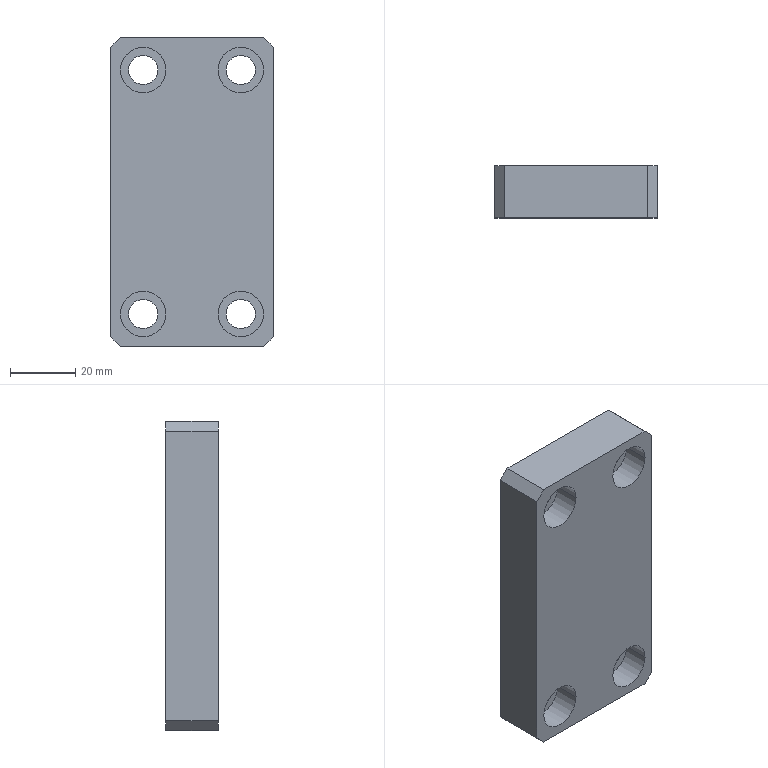Component | SolidWorks | -LowerStopBlock-1 | 1 solid | 30 faces | box 50 x 16 x 95 mm | volume 68750 mm3 | cylinder 16 | plane 14 | commonest cylinder face diameters 14 x8 9 x8
build123d program:
from build123d import *

# Parameters (mm, degrees)
SKETCH1_W                                         = 95
SKETCH1_H                                         = 50
BOSS_EXTRUDE1_DEPTH                               = 8
HOLE_SIZE_ACCORDING_TO_SLOTTED_PAN_HE_D           = 9
HOLE_SIZE_ACCORDING_TO_SLOTTED_PAN_HE_CBORE_D     = 14
HOLE_SIZE_ACCORDING_TO_SLOTTED_PAN_HE_CBORE_DEPTH = 8
CHAMFER1_SIZE                                     = 3


with BuildPart() as part:
    # Sketch1 → Boss-Extrude1 (new, symmetric)
    with BuildSketch(Plane(origin=(0, 0, 0), x_dir=(1, 0, 0), z_dir=(0, 1, 0))):
        Rectangle(SKETCH1_W, SKETCH1_H)
    extrude(amount=BOSS_EXTRUDE1_DEPTH, both=True)

    # Hole Size _ according to_ Slotted Pan He (through all)
    with Locations(Plane(origin=(0, 8, 0), x_dir=(1, 0, 0), z_dir=(0, 1, 0))):
        with Locations((-37.5, 15), (-37.5, -15), (37.5, 15), (37.5, -15)):
            CounterBoreHole(HOLE_SIZE_ACCORDING_TO_SLOTTED_PAN_HE_D / 2, HOLE_SIZE_ACCORDING_TO_SLOTTED_PAN_HE_CBORE_D / 2, HOLE_SIZE_ACCORDING_TO_SLOTTED_PAN_HE_CBORE_DEPTH)

    # Chamfer1
    chamfer1_edges = [part.edges().sort_by_distance(p)[0] for p in [
        (-47.5, 0, -25),
        (47.5, 0, -25),
        (47.5, 0, 25),
        (-47.5, 0, 25),
    ]]
    chamfer(chamfer1_edges, length=CHAMFER1_SIZE)


solid = part.part

# Placed as in the assembly
solid = solid.moved(Location((30, 1036.5, -40), (180, 90, 0)))
STEP:
#1=CARTESIAN_POINT('',(2.047,40.807,-0.09843));
#2=VERTEX_POINT('',#1);
#3=CARTESIAN_POINT('',(1.496,40.807,-0.09843));
#4=VERTEX_POINT('',#3);
#5=CARTESIAN_POINT('',(1.772,40.807,-0.09843));
#6=DIRECTION('',(0.,-1.,0.));
#7=DIRECTION('',(-1.,0.,-0.));
#8=AXIS2_PLACEMENT_3D('',#5,#6,#7);
#9=CIRCLE('',#8,0.2756);
#10=EDGE_CURVE('',#2,#4,#9,.T.);
#11=ORIENTED_EDGE('',*,*,#10,.F.);
#12=CARTESIAN_POINT('',(2.047,40.492,-0.09843));
#13=VERTEX_POINT('',#12);
#14=CARTESIAN_POINT('',(2.047,40.492,-0.09843));
#15=DIRECTION('',(0.,-1.,0.));
#16=VECTOR('',#15,39.37);
#17=LINE('',#14,#16);
#18=EDGE_CURVE('',#2,#13,#17,.T.);
#19=ORIENTED_EDGE('',*,*,#18,.T.);
#20=CARTESIAN_POINT('',(1.496,40.492,-0.09843));
#21=VERTEX_POINT('',#20);
#22=CARTESIAN_POINT('',(1.772,40.492,-0.09843));
#23=DIRECTION('',(0.,-1.,0.));
#24=DIRECTION('',(-1.,0.,-0.));
#25=AXIS2_PLACEMENT_3D('',#22,#23,#24);
#26=CIRCLE('',#25,0.2756);
#27=EDGE_CURVE('',#13,#21,#26,.T.);
#28=ORIENTED_EDGE('',*,*,#27,.T.);
#29=CARTESIAN_POINT('',(1.496,40.492,-0.09843));
#30=DIRECTION('',(0.,-1.,0.));
#31=VECTOR('',#30,39.37);
#32=LINE('',#29,#31);
#33=EDGE_CURVE('',#4,#21,#32,.T.);
#34=ORIENTED_EDGE('',*,*,#33,.F.);
#35=EDGE_LOOP('',(#11,#19,#28,#34));
#36=FACE_OUTER_BOUND('',#35,.T.);
#37=CARTESIAN_POINT('',(1.772,40.492,-0.09843));
#38=DIRECTION('',(0.,-1.,0.));
#39=DIRECTION('',(-1.,0.,-0.));
#40=AXIS2_PLACEMENT_3D('',#37,#38,#39);
#41=CYLINDRICAL_SURFACE('',#40,0.2756);
#42=ADVANCED_FACE('',(#36),#41,.F.);
#43=CARTESIAN_POINT('',(1.949,41.122,-0.09843));
#44=VERTEX_POINT('',#43);
#45=CARTESIAN_POINT('',(1.594,41.122,-0.09843));
#46=VERTEX_POINT('',#45);
#47=CARTESIAN_POINT('',(1.772,41.122,-0.09843));
#48=DIRECTION('',(0.,-1.,0.));
#49=DIRECTION('',(-1.,0.,-0.));
#50=AXIS2_PLACEMENT_3D('',#47,#48,#49);
#51=CIRCLE('',#50,0.1772);
#52=EDGE_CURVE('',#44,#46,#51,.T.);
#53=ORIENTED_EDGE('',*,*,#52,.F.);
#54=CARTESIAN_POINT('',(1.949,40.807,-0.09843));
#55=VERTEX_POINT('',#54);
#56=CARTESIAN_POINT('',(1.949,40.492,-0.09843));
#57=DIRECTION('',(0.,-1.,0.));
#58=VECTOR('',#57,39.37);
#59=LINE('',#56,#58);
#60=EDGE_CURVE('',#44,#55,#59,.T.);
#61=ORIENTED_EDGE('',*,*,#60,.T.);
#62=CARTESIAN_POINT('',(1.594,40.807,-0.09843));
#63=VERTEX_POINT('',#62);
#64=CARTESIAN_POINT('',(1.772,40.807,-0.09843));
#65=DIRECTION('',(0.,-1.,0.));
#66=DIRECTION('',(-1.,0.,-0.));
#67=AXIS2_PLACEMENT_3D('',#64,#65,#66);
#68=CIRCLE('',#67,0.1772);
#69=EDGE_CURVE('',#55,#63,#68,.T.);
#70=ORIENTED_EDGE('',*,*,#69,.T.);
#71=CARTESIAN_POINT('',(1.594,40.492,-0.09843));
#72=DIRECTION('',(0.,-1.,0.));
#73=VECTOR('',#72,39.37);
#74=LINE('',#71,#73);
#75=EDGE_CURVE('',#46,#63,#74,.T.);
#76=ORIENTED_EDGE('',*,*,#75,.F.);
#77=EDGE_LOOP('',(#53,#61,#70,#76));
#78=FACE_OUTER_BOUND('',#77,.T.);
#79=CARTESIAN_POINT('',(1.772,40.492,-0.09843));
#80=DIRECTION('',(0.,-1.,0.));
#81=DIRECTION('',(-1.,0.,-0.));
#82=AXIS2_PLACEMENT_3D('',#79,#80,#81);
#83=CYLINDRICAL_SURFACE('',#82,0.1772);
#84=ADVANCED_FACE('',(#78),#83,.F.);
#85=CARTESIAN_POINT('',(0.8661,40.807,-0.09843));
#86=VERTEX_POINT('',#85);
#87=CARTESIAN_POINT('',(0.315,40.807,-0.09843));
#88=VERTEX_POINT('',#87);
#89=CARTESIAN_POINT('',(0.5906,40.807,-0.09843));
#90=DIRECTION('',(0.,-1.,0.));
#91=DIRECTION('',(-1.,0.,-0.));
#92=AXIS2_PLACEMENT_3D('',#89,#90,#91);
#93=CIRCLE('',#92,0.2756);
#94=EDGE_CURVE('',#86,#88,#93,.T.);
#95=ORIENTED_EDGE('',*,*,#94,.F.);
#96=CARTESIAN_POINT('',(0.8661,40.492,-0.09843));
#97=VERTEX_POINT('',#96);
#98=CARTESIAN_POINT('',(0.8661,40.492,-0.09843));
#99=DIRECTION('',(0.,-1.,0.));
#100=VECTOR('',#99,39.37);
#101=LINE('',#98,#100);
#102=EDGE_CURVE('',#86,#97,#101,.T.);
#103=ORIENTED_EDGE('',*,*,#102,.T.);
#104=CARTESIAN_POINT('',(0.315,40.492,-0.09843));
#105=VERTEX_POINT('',#104);
#106=CARTESIAN_POINT('',(0.5906,40.492,-0.09843));
#107=DIRECTION('',(0.,-1.,0.));
#108=DIRECTION('',(-1.,0.,-0.));
#109=AXIS2_PLACEMENT_3D('',#106,#107,#108);
#110=CIRCLE('',#109,0.2756);
#111=EDGE_CURVE('',#97,#105,#110,.T.);
#112=ORIENTED_EDGE('',*,*,#111,.T.);
#113=CARTESIAN_POINT('',(0.315,40.492,-0.09843));
#114=DIRECTION('',(0.,-1.,0.));
#115=VECTOR('',#114,39.37);
#116=LINE('',#113,#115);
#117=EDGE_CURVE('',#88,#105,#116,.T.);
#118=ORIENTED_EDGE('',*,*,#117,.F.);
#119=EDGE_LOOP('',(#95,#103,#112,#118));
#120=FACE_OUTER_BOUND('',#119,.T.);
#121=CARTESIAN_POINT('',(0.5906,40.492,-0.09843));
#122=DIRECTION('',(0.,-1.,0.));
#123=DIRECTION('',(-1.,0.,-0.));
#124=AXIS2_PLACEMENT_3D('',#121,#122,#123);
#125=CYLINDRICAL_SURFACE('',#124,0.2756);
#126=ADVANCED_FACE('',(#120),#125,.F.);
#127=CARTESIAN_POINT('',(0.7677,41.122,-0.09843));
#128=VERTEX_POINT('',#127);
#129=CARTESIAN_POINT('',(0.4134,41.122,-0.09843));
#130=VERTEX_POINT('',#129);
#131=CARTESIAN_POINT('',(0.5906,41.122,-0.09843));
#132=DIRECTION('',(0.,-1.,0.));
#133=DIRECTION('',(-1.,0.,-0.));
#134=AXIS2_PLACEMENT_3D('',#131,#132,#133);
#135=CIRCLE('',#134,0.1772);
#136=EDGE_CURVE('',#128,#130,#135,.T.);
#137=ORIENTED_EDGE('',*,*,#136,.F.);
#138=CARTESIAN_POINT('',(0.7677,40.807,-0.09843));
#139=VERTEX_POINT('',#138);
#140=CARTESIAN_POINT('',(0.7677,40.492,-0.09843));
#141=DIRECTION('',(0.,-1.,0.));
#142=VECTOR('',#141,39.37);
#143=LINE('',#140,#142);
#144=EDGE_CURVE('',#128,#139,#143,.T.);
#145=ORIENTED_EDGE('',*,*,#144,.T.);
#146=CARTESIAN_POINT('',(0.4134,40.807,-0.09843));
#147=VERTEX_POINT('',#146);
#148=CARTESIAN_POINT('',(0.5906,40.807,-0.09843));
#149=DIRECTION('',(0.,-1.,0.));
#150=DIRECTION('',(-1.,0.,-0.));
#151=AXIS2_PLACEMENT_3D('',#148,#149,#150);
#152=CIRCLE('',#151,0.1772);
#153=EDGE_CURVE('',#139,#147,#152,.T.);
#154=ORIENTED_EDGE('',*,*,#153,.T.);
#155=CARTESIAN_POINT('',(0.4134,40.492,-0.09843));
#156=DIRECTION('',(0.,-1.,0.));
#157=VECTOR('',#156,39.37);
#158=LINE('',#155,#157);
#159=EDGE_CURVE('',#130,#147,#158,.T.);
#160=ORIENTED_EDGE('',*,*,#159,.F.);
#161=EDGE_LOOP('',(#137,#145,#154,#160));
#162=FACE_OUTER_BOUND('',#161,.T.);
#163=CARTESIAN_POINT('',(0.5906,40.492,-0.09843));
#164=DIRECTION('',(0.,-1.,0.));
#165=DIRECTION('',(-1.,0.,-0.));
#166=AXIS2_PLACEMENT_3D('',#163,#164,#165);
#167=CYLINDRICAL_SURFACE('',#166,0.1772);
#168=ADVANCED_FACE('',(#162),#167,.F.);
#169=CARTESIAN_POINT('',(2.047,40.807,-3.051));
#170=VERTEX_POINT('',#169);
#171=CARTESIAN_POINT('',(1.496,40.807,-3.051));
#172=VERTEX_POINT('',#171);
#173=CARTESIAN_POINT('',(1.772,40.807,-3.051));
#174=DIRECTION('',(0.,-1.,0.));
#175=DIRECTION('',(-1.,0.,0.));
#176=AXIS2_PLACEMENT_3D('',#173,#174,#175);
#177=CIRCLE('',#176,0.2756);
#178=EDGE_CURVE('',#170,#172,#177,.T.);
#179=ORIENTED_EDGE('',*,*,#178,.F.);
#180=CARTESIAN_POINT('',(2.047,40.492,-3.051));
#181=VERTEX_POINT('',#180);
#182=CARTESIAN_POINT('',(2.047,40.492,-3.051));
#183=DIRECTION('',(0.,-1.,0.));
#184=VECTOR('',#183,39.37);
#185=LINE('',#182,#184);
#186=EDGE_CURVE('',#170,#181,#185,.T.);
#187=ORIENTED_EDGE('',*,*,#186,.T.);
#188=CARTESIAN_POINT('',(1.496,40.492,-3.051));
#189=VERTEX_POINT('',#188);
#190=CARTESIAN_POINT('',(1.772,40.492,-3.051));
#191=DIRECTION('',(0.,-1.,0.));
#192=DIRECTION('',(-1.,0.,0.));
#193=AXIS2_PLACEMENT_3D('',#190,#191,#192);
#194=CIRCLE('',#193,0.2756);
#195=EDGE_CURVE('',#181,#189,#194,.T.);
#196=ORIENTED_EDGE('',*,*,#195,.T.);
#197=CARTESIAN_POINT('',(1.496,40.492,-3.051));
#198=DIRECTION('',(0.,-1.,0.));
#199=VECTOR('',#198,39.37);
#200=LINE('',#197,#199);
#201=EDGE_CURVE('',#172,#189,#200,.T.);
#202=ORIENTED_EDGE('',*,*,#201,.F.);
#203=EDGE_LOOP('',(#179,#187,#196,#202));
#204=FACE_OUTER_BOUND('',#203,.T.);
#205=CARTESIAN_POINT('',(1.772,40.492,-3.051));
#206=DIRECTION('',(0.,-1.,0.));
#207=DIRECTION('',(-1.,0.,0.));
#208=AXIS2_PLACEMENT_3D('',#205,#206,#207);
#209=CYLINDRICAL_SURFACE('',#208,0.2756);
#210=ADVANCED_FACE('',(#204),#209,.F.);
#211=CARTESIAN_POINT('',(1.949,41.122,-3.051));
#212=VERTEX_POINT('',#211);
#213=CARTESIAN_POINT('',(1.594,41.122,-3.051));
#214=VERTEX_POINT('',#213);
#215=CARTESIAN_POINT('',(1.772,41.122,-3.051));
#216=DIRECTION('',(0.,-1.,0.));
#217=DIRECTION('',(-1.,0.,0.));
#218=AXIS2_PLACEMENT_3D('',#215,#216,#217);
#219=CIRCLE('',#218,0.1772);
#220=EDGE_CURVE('',#212,#214,#219,.T.);
#221=ORIENTED_EDGE('',*,*,#220,.F.);
#222=CARTESIAN_POINT('',(1.949,40.807,-3.051));
#223=VERTEX_POINT('',#222);
#224=CARTESIAN_POINT('',(1.949,40.492,-3.051));
#225=DIRECTION('',(0.,-1.,0.));
#226=VECTOR('',#225,39.37);
#227=LINE('',#224,#226);
#228=EDGE_CURVE('',#212,#223,#227,.T.);
#229=ORIENTED_EDGE('',*,*,#228,.T.);
#230=CARTESIAN_POINT('',(1.594,40.807,-3.051));
#231=VERTEX_POINT('',#230);
#232=CARTESIAN_POINT('',(1.772,40.807,-3.051));
#233=DIRECTION('',(0.,-1.,0.));
#234=DIRECTION('',(-1.,0.,0.));
#235=AXIS2_PLACEMENT_3D('',#232,#233,#234);
#236=CIRCLE('',#235,0.1772);
#237=EDGE_CURVE('',#223,#231,#236,.T.);
#238=ORIENTED_EDGE('',*,*,#237,.T.);
#239=CARTESIAN_POINT('',(1.594,40.492,-3.051));
#240=DIRECTION('',(0.,-1.,0.));
#241=VECTOR('',#240,39.37);
#242=LINE('',#239,#241);
#243=EDGE_CURVE('',#214,#231,#242,.T.);
#244=ORIENTED_EDGE('',*,*,#243,.F.);
#245=EDGE_LOOP('',(#221,#229,#238,#244));
#246=FACE_OUTER_BOUND('',#245,.T.);
#247=CARTESIAN_POINT('',(1.772,40.492,-3.051));
#248=DIRECTION('',(0.,-1.,0.));
#249=DIRECTION('',(-1.,0.,0.));
#250=AXIS2_PLACEMENT_3D('',#247,#248,#249);
#251=CYLINDRICAL_SURFACE('',#250,0.1772);
#252=ADVANCED_FACE('',(#246),#251,.F.);
#253=CARTESIAN_POINT('',(0.8661,40.807,-3.051));
#254=VERTEX_POINT('',#253);
#255=CARTESIAN_POINT('',(0.315,40.807,-3.051));
#256=VERTEX_POINT('',#255);
#257=CARTESIAN_POINT('',(0.5906,40.807,-3.051));
#258=DIRECTION('',(0.,-1.,0.));
#259=DIRECTION('',(-1.,0.,0.));
#260=AXIS2_PLACEMENT_3D('',#257,#258,#259);
#261=CIRCLE('',#260,0.2756);
#262=EDGE_CURVE('',#254,#256,#261,.T.);
#263=ORIENTED_EDGE('',*,*,#262,.F.);
#264=CARTESIAN_POINT('',(0.8661,40.492,-3.051));
#265=VERTEX_POINT('',#264);
#266=CARTESIAN_POINT('',(0.8661,40.492,-3.051));
#267=DIRECTION('',(0.,-1.,0.));
#268=VECTOR('',#267,39.37);
#269=LINE('',#266,#268);
#270=EDGE_CURVE('',#254,#265,#269,.T.);
#271=ORIENTED_EDGE('',*,*,#270,.T.);
#272=CARTESIAN_POINT('',(0.315,40.492,-3.051));
#273=VERTEX_POINT('',#272);
#274=CARTESIAN_POINT('',(0.5906,40.492,-3.051));
#275=DIRECTION('',(0.,-1.,0.));
#276=DIRECTION('',(-1.,0.,0.));
#277=AXIS2_PLACEMENT_3D('',#274,#275,#276);
#278=CIRCLE('',#277,0.2756);
#279=EDGE_CURVE('',#265,#273,#278,.T.);
#280=ORIENTED_EDGE('',*,*,#279,.T.);
#281=CARTESIAN_POINT('',(0.315,40.492,-3.051));
#282=DIRECTION('',(0.,-1.,0.));
#283=VECTOR('',#282,39.37);
#284=LINE('',#281,#283);
#285=EDGE_CURVE('',#256,#273,#284,.T.);
#286=ORIENTED_EDGE('',*,*,#285,.F.);
#287=EDGE_LOOP('',(#263,#271,#280,#286));
#288=FACE_OUTER_BOUND('',#287,.T.);
#289=CARTESIAN_POINT('',(0.5906,40.492,-3.051));
#290=DIRECTION('',(0.,-1.,0.));
#291=DIRECTION('',(-1.,0.,0.));
#292=AXIS2_PLACEMENT_3D('',#289,#290,#291);
#293=CYLINDRICAL_SURFACE('',#292,0.2756);
#294=ADVANCED_FACE('',(#288),#293,.F.);
#295=CARTESIAN_POINT('',(0.7677,41.122,-3.051));
#296=VERTEX_POINT('',#295);
#297=CARTESIAN_POINT('',(0.4134,41.122,-3.051));
#298=VERTEX_POINT('',#297);
#299=CARTESIAN_POINT('',(0.5906,41.122,-3.051));
#300=DIRECTION('',(0.,-1.,0.));
#301=DIRECTION('',(-1.,0.,0.));
#302=AXIS2_PLACEMENT_3D('',#299,#300,#301);
#303=CIRCLE('',#302,0.1772);
#304=EDGE_CURVE('',#296,#298,#303,.T.);
#305=ORIENTED_EDGE('',*,*,#304,.F.);
#306=CARTESIAN_POINT('',(0.7677,40.807,-3.051));
#307=VERTEX_POINT('',#306);
#308=CARTESIAN_POINT('',(0.7677,40.492,-3.051));
#309=DIRECTION('',(0.,-1.,0.));
#310=VECTOR('',#309,39.37);
#311=LINE('',#308,#310);
#312=EDGE_CURVE('',#296,#307,#311,.T.);
#313=ORIENTED_EDGE('',*,*,#312,.T.);
#314=CARTESIAN_POINT('',(0.4134,40.807,-3.051));
#315=VERTEX_POINT('',#314);
#316=CARTESIAN_POINT('',(0.5906,40.807,-3.051));
#317=DIRECTION('',(0.,-1.,0.));
#318=DIRECTION('',(-1.,0.,0.));
#319=AXIS2_PLACEMENT_3D('',#316,#317,#318);
#320=CIRCLE('',#319,0.1772);
#321=EDGE_CURVE('',#307,#315,#320,.T.);
#322=ORIENTED_EDGE('',*,*,#321,.T.);
#323=CARTESIAN_POINT('',(0.4134,40.492,-3.051));
#324=DIRECTION('',(0.,-1.,0.));
#325=VECTOR('',#324,39.37);
#326=LINE('',#323,#325);
#327=EDGE_CURVE('',#298,#315,#326,.T.);
#328=ORIENTED_EDGE('',*,*,#327,.F.);
#329=EDGE_LOOP('',(#305,#313,#322,#328));
#330=FACE_OUTER_BOUND('',#329,.T.);
#331=CARTESIAN_POINT('',(0.5906,40.492,-3.051));
#332=DIRECTION('',(0.,-1.,0.));
#333=DIRECTION('',(-1.,0.,0.));
#334=AXIS2_PLACEMENT_3D('',#331,#332,#333);
#335=CYLINDRICAL_SURFACE('',#334,0.1772);
#336=ADVANCED_FACE('',(#330),#335,.F.);
#337=CARTESIAN_POINT('',(2.047,40.492,0.2953));
#338=VERTEX_POINT('',#337);
#339=CARTESIAN_POINT('',(0.315,40.492,0.2953));
#340=VERTEX_POINT('',#339);
#341=CARTESIAN_POINT('',(0.1969,40.492,0.2953));
#342=DIRECTION('',(-1.,0.,-0.));
#343=VECTOR('',#342,39.37);
#344=LINE('',#341,#343);
#345=EDGE_CURVE('',#338,#340,#344,.T.);
#346=ORIENTED_EDGE('',*,*,#345,.F.);
#347=CARTESIAN_POINT('',(2.047,41.122,0.2953));
#348=VERTEX_POINT('',#347);
#349=CARTESIAN_POINT('',(2.047,40.492,0.2953));
#350=DIRECTION('',(0.,1.,0.));
#351=VECTOR('',#350,39.37);
#352=LINE('',#349,#351);
#353=EDGE_CURVE('',#338,#348,#352,.T.);
#354=ORIENTED_EDGE('',*,*,#353,.T.);
#355=CARTESIAN_POINT('',(0.315,41.122,0.2953));
#356=VERTEX_POINT('',#355);
#357=CARTESIAN_POINT('',(0.1969,41.122,0.2953));
#358=DIRECTION('',(-1.,0.,-0.));
#359=VECTOR('',#358,39.37);
#360=LINE('',#357,#359);
#361=EDGE_CURVE('',#348,#356,#360,.T.);
#362=ORIENTED_EDGE('',*,*,#361,.T.);
#363=CARTESIAN_POINT('',(0.315,40.492,0.2953));
#364=DIRECTION('',(0.,-1.,0.));
#365=VECTOR('',#364,39.37);
#366=LINE('',#363,#365);
#367=EDGE_CURVE('',#356,#340,#366,.T.);
#368=ORIENTED_EDGE('',*,*,#367,.T.);
#369=EDGE_LOOP('',(#346,#354,#362,#368));
#370=FACE_OUTER_BOUND('',#369,.T.);
#371=CARTESIAN_POINT('',(0.1969,40.492,0.2953));
#372=DIRECTION('',(0.,0.,-1.));
#373=DIRECTION('',(1.,0.,0.));
#374=AXIS2_PLACEMENT_3D('',#371,#372,#373);
#375=PLANE('',#374);
#376=ADVANCED_FACE('',(#370),#375,.F.);
#377=CARTESIAN_POINT('',(0.1969,41.122,0.1772));
#378=VERTEX_POINT('',#377);
#379=CARTESIAN_POINT('',(0.1969,41.122,-3.327));
#380=VERTEX_POINT('',#379);
#381=CARTESIAN_POINT('',(0.1969,41.122,-3.445));
#382=DIRECTION('',(0.,0.,-1.));
#383=VECTOR('',#382,39.37);
#384=LINE('',#381,#383);
#385=EDGE_CURVE('',#378,#380,#384,.T.);
#386=ORIENTED_EDGE('',*,*,#385,.T.);
#387=CARTESIAN_POINT('',(0.1969,40.492,-3.327));
#388=VERTEX_POINT('',#387);
#389=CARTESIAN_POINT('',(0.1969,40.492,-3.327));
#390=DIRECTION('',(0.,-1.,0.));
#391=VECTOR('',#390,39.37);
#392=LINE('',#389,#391);
#393=EDGE_CURVE('',#380,#388,#392,.T.);
#394=ORIENTED_EDGE('',*,*,#393,.T.);
#395=CARTESIAN_POINT('',(0.1969,40.492,0.1772));
#396=VERTEX_POINT('',#395);
#397=CARTESIAN_POINT('',(0.1969,40.492,-3.445));
#398=DIRECTION('',(0.,0.,-1.));
#399=VECTOR('',#398,39.37);
#400=LINE('',#397,#399);
#401=EDGE_CURVE('',#396,#388,#400,.T.);
#402=ORIENTED_EDGE('',*,*,#401,.F.);
#403=CARTESIAN_POINT('',(0.1969,40.492,0.1772));
#404=DIRECTION('',(0.,1.,0.));
#405=VECTOR('',#404,39.37);
#406=LINE('',#403,#405);
#407=EDGE_CURVE('',#396,#378,#406,.T.);
#408=ORIENTED_EDGE('',*,*,#407,.T.);
#409=EDGE_LOOP('',(#386,#394,#402,#408));
#410=FACE_OUTER_BOUND('',#409,.T.);
#411=CARTESIAN_POINT('',(0.1969,40.492,-3.445));
#412=DIRECTION('',(1.,0.,0.));
#413=DIRECTION('',(-0.,0.,1.));
#414=AXIS2_PLACEMENT_3D('',#411,#412,#413);
#415=PLANE('',#414);
#416=ADVANCED_FACE('',(#410),#415,.F.);
#417=CARTESIAN_POINT('',(0.315,40.492,-3.445));
#418=VERTEX_POINT('',#417);
#419=CARTESIAN_POINT('',(2.047,40.492,-3.445));
#420=VERTEX_POINT('',#419);
#421=CARTESIAN_POINT('',(0.1969,40.492,-3.445));
#422=DIRECTION('',(1.,0.,0.));
#423=VECTOR('',#422,39.37);
#424=LINE('',#421,#423);
#425=EDGE_CURVE('',#418,#420,#424,.T.);
#426=ORIENTED_EDGE('',*,*,#425,.F.);
#427=CARTESIAN_POINT('',(0.315,41.122,-3.445));
#428=VERTEX_POINT('',#427);
#429=CARTESIAN_POINT('',(0.315,40.492,-3.445));
#430=DIRECTION('',(0.,1.,0.));
#431=VECTOR('',#430,39.37);
#432=LINE('',#429,#431);
#433=EDGE_CURVE('',#418,#428,#432,.T.);
#434=ORIENTED_EDGE('',*,*,#433,.T.);
#435=CARTESIAN_POINT('',(2.047,41.122,-3.445));
#436=VERTEX_POINT('',#435);
#437=CARTESIAN_POINT('',(0.1969,41.122,-3.445));
#438=DIRECTION('',(1.,0.,0.));
#439=VECTOR('',#438,39.37);
#440=LINE('',#437,#439);
#441=EDGE_CURVE('',#428,#436,#440,.T.);
#442=ORIENTED_EDGE('',*,*,#441,.T.);
#443=CARTESIAN_POINT('',(2.047,40.492,-3.445));
#444=DIRECTION('',(0.,-1.,0.));
#445=VECTOR('',#444,39.37);
#446=LINE('',#443,#445);
#447=EDGE_CURVE('',#436,#420,#446,.T.);
#448=ORIENTED_EDGE('',*,*,#447,.T.);
#449=EDGE_LOOP('',(#426,#434,#442,#448));
#450=FACE_OUTER_BOUND('',#449,.T.);
#451=CARTESIAN_POINT('',(0.1969,40.492,-3.445));
#452=DIRECTION('',(-0.,0.,1.));
#453=DIRECTION('',(-1.,0.,-0.));
#454=AXIS2_PLACEMENT_3D('',#451,#452,#453);
#455=PLANE('',#454);
#456=ADVANCED_FACE('',(#450),#455,.F.);
#457=CARTESIAN_POINT('',(2.165,40.492,-3.327));
#458=VERTEX_POINT('',#457);
#459=CARTESIAN_POINT('',(2.165,40.492,0.1772));
#460=VERTEX_POINT('',#459);
#461=CARTESIAN_POINT('',(2.165,40.492,-3.445));
#462=DIRECTION('',(-0.,0.,1.));
#463=VECTOR('',#462,39.37);
#464=LINE('',#461,#463);
#465=EDGE_CURVE('',#458,#460,#464,.T.);
#466=ORIENTED_EDGE('',*,*,#465,.F.);
#467=CARTESIAN_POINT('',(2.165,41.122,-3.327));
#468=VERTEX_POINT('',#467);
#469=CARTESIAN_POINT('',(2.165,40.492,-3.327));
#470=DIRECTION('',(0.,1.,0.));
#471=VECTOR('',#470,39.37);
#472=LINE('',#469,#471);
#473=EDGE_CURVE('',#458,#468,#472,.T.);
#474=ORIENTED_EDGE('',*,*,#473,.T.);
#475=CARTESIAN_POINT('',(2.165,41.122,0.1772));
#476=VERTEX_POINT('',#475);
#477=CARTESIAN_POINT('',(2.165,41.122,-3.445));
#478=DIRECTION('',(-0.,0.,1.));
#479=VECTOR('',#478,39.37);
#480=LINE('',#477,#479);
#481=EDGE_CURVE('',#468,#476,#480,.T.);
#482=ORIENTED_EDGE('',*,*,#481,.T.);
#483=CARTESIAN_POINT('',(2.165,40.492,0.1772));
#484=DIRECTION('',(0.,-1.,0.));
#485=VECTOR('',#484,39.37);
#486=LINE('',#483,#485);
#487=EDGE_CURVE('',#476,#460,#486,.T.);
#488=ORIENTED_EDGE('',*,*,#487,.T.);
#489=EDGE_LOOP('',(#466,#474,#482,#488));
#490=FACE_OUTER_BOUND('',#489,.T.);
#491=CARTESIAN_POINT('',(2.165,40.492,-3.445));
#492=DIRECTION('',(-1.,0.,-0.));
#493=DIRECTION('',(0.,0.,-1.));
#494=AXIS2_PLACEMENT_3D('',#491,#492,#493);
#495=PLANE('',#494);
#496=ADVANCED_FACE('',(#490),#495,.F.);
#497=CARTESIAN_POINT('',(1.772,40.492,-0.09843));
#498=DIRECTION('',(0.,-1.,0.));
#499=DIRECTION('',(-1.,0.,-0.));
#500=AXIS2_PLACEMENT_3D('',#497,#498,#499);
#501=CIRCLE('',#500,0.2756);
#502=EDGE_CURVE('',#21,#13,#501,.T.);
#503=ORIENTED_EDGE('',*,*,#502,.F.);
#504=ORIENTED_EDGE('',*,*,#27,.F.);
#505=EDGE_LOOP('',(#503,#504));
#506=FACE_BOUND('',#505,.T.);
#507=CARTESIAN_POINT('',(0.5906,40.492,-0.09843));
#508=DIRECTION('',(0.,-1.,0.));
#509=DIRECTION('',(-1.,0.,-0.));
#510=AXIS2_PLACEMENT_3D('',#507,#508,#509);
#511=CIRCLE('',#510,0.2756);
#512=EDGE_CURVE('',#105,#97,#511,.T.);
#513=ORIENTED_EDGE('',*,*,#512,.F.);
#514=ORIENTED_EDGE('',*,*,#111,.F.);
#515=EDGE_LOOP('',(#513,#514));
#516=FACE_BOUND('',#515,.T.);
#517=CARTESIAN_POINT('',(1.772,40.492,-3.051));
#518=DIRECTION('',(0.,-1.,0.));
#519=DIRECTION('',(-1.,0.,0.));
#520=AXIS2_PLACEMENT_3D('',#517,#518,#519);
#521=CIRCLE('',#520,0.2756);
#522=EDGE_CURVE('',#189,#181,#521,.T.);
#523=ORIENTED_EDGE('',*,*,#522,.F.);
#524=ORIENTED_EDGE('',*,*,#195,.F.);
#525=EDGE_LOOP('',(#523,#524));
#526=FACE_BOUND('',#525,.T.);
#527=CARTESIAN_POINT('',(0.5906,40.492,-3.051));
#528=DIRECTION('',(0.,-1.,0.));
#529=DIRECTION('',(-1.,0.,0.));
#530=AXIS2_PLACEMENT_3D('',#527,#528,#529);
#531=CIRCLE('',#530,0.2756);
#532=EDGE_CURVE('',#273,#265,#531,.T.);
#533=ORIENTED_EDGE('',*,*,#532,.F.);
#534=ORIENTED_EDGE('',*,*,#279,.F.);
#535=EDGE_LOOP('',(#533,#534));
#536=FACE_BOUND('',#535,.T.);
#537=ORIENTED_EDGE('',*,*,#401,.T.);
#538=CARTESIAN_POINT('',(-0.187,40.492,-2.943));
#539=DIRECTION('',(0.7071,0.,-0.7071));
#540=VECTOR('',#539,39.37);
#541=LINE('',#538,#540);
#542=EDGE_CURVE('',#388,#418,#541,.T.);
#543=ORIENTED_EDGE('',*,*,#542,.T.);
#544=ORIENTED_EDGE('',*,*,#425,.T.);
#545=CARTESIAN_POINT('',(2.549,40.492,-2.943));
#546=DIRECTION('',(0.7071,0.,0.7071));
#547=VECTOR('',#546,39.37);
#548=LINE('',#545,#547);
#549=EDGE_CURVE('',#420,#458,#548,.T.);
#550=ORIENTED_EDGE('',*,*,#549,.T.);
#551=ORIENTED_EDGE('',*,*,#465,.T.);
#552=CARTESIAN_POINT('',(2.549,40.492,-0.2067));
#553=DIRECTION('',(-0.7071,0.,0.7071));
#554=VECTOR('',#553,39.37);
#555=LINE('',#552,#554);
#556=EDGE_CURVE('',#460,#338,#555,.T.);
#557=ORIENTED_EDGE('',*,*,#556,.T.);
#558=ORIENTED_EDGE('',*,*,#345,.T.);
#559=CARTESIAN_POINT('',(-0.187,40.492,-0.2067));
#560=DIRECTION('',(-0.7071,0.,-0.7071));
#561=VECTOR('',#560,39.37);
#562=LINE('',#559,#561);
#563=EDGE_CURVE('',#340,#396,#562,.T.);
#564=ORIENTED_EDGE('',*,*,#563,.T.);
#565=EDGE_LOOP('',(#537,#543,#544,#550,#551,#557,#558,#564));
#566=FACE_OUTER_BOUND('',#565,.T.);
#567=CARTESIAN_POINT('',(1.181,40.492,-1.575));
#568=DIRECTION('',(0.,-1.,0.));
#569=DIRECTION('',(-1.,0.,-0.));
#570=AXIS2_PLACEMENT_3D('',#567,#568,#569);
#571=PLANE('',#570);
#572=ADVANCED_FACE('',(#506,#516,#526,#536,#566),#571,.T.);
#573=CARTESIAN_POINT('',(1.772,41.122,-0.09843));
#574=DIRECTION('',(0.,-1.,0.));
#575=DIRECTION('',(-1.,0.,-0.));
#576=AXIS2_PLACEMENT_3D('',#573,#574,#575);
#577=CIRCLE('',#576,0.1772);
#578=EDGE_CURVE('',#46,#44,#577,.T.);
#579=ORIENTED_EDGE('',*,*,#578,.T.);
#580=ORIENTED_EDGE('',*,*,#52,.T.);
#581=EDGE_LOOP('',(#579,#580));
#582=FACE_BOUND('',#581,.T.);
#583=CARTESIAN_POINT('',(0.5906,41.122,-0.09843));
#584=DIRECTION('',(0.,-1.,0.));
#585=DIRECTION('',(-1.,0.,-0.));
#586=AXIS2_PLACEMENT_3D('',#583,#584,#585);
#587=CIRCLE('',#586,0.1772);
#588=EDGE_CURVE('',#130,#128,#587,.T.);
#589=ORIENTED_EDGE('',*,*,#588,.T.);
#590=ORIENTED_EDGE('',*,*,#136,.T.);
#591=EDGE_LOOP('',(#589,#590));
#592=FACE_BOUND('',#591,.T.);
#593=CARTESIAN_POINT('',(1.772,41.122,-3.051));
#594=DIRECTION('',(0.,-1.,0.));
#595=DIRECTION('',(-1.,0.,0.));
#596=AXIS2_PLACEMENT_3D('',#593,#594,#595);
#597=CIRCLE('',#596,0.1772);
#598=EDGE_CURVE('',#214,#212,#597,.T.);
#599=ORIENTED_EDGE('',*,*,#598,.T.);
#600=ORIENTED_EDGE('',*,*,#220,.T.);
#601=EDGE_LOOP('',(#599,#600));
#602=FACE_BOUND('',#601,.T.);
#603=CARTESIAN_POINT('',(0.5906,41.122,-3.051));
#604=DIRECTION('',(0.,-1.,0.));
#605=DIRECTION('',(-1.,0.,0.));
#606=AXIS2_PLACEMENT_3D('',#603,#604,#605);
#607=CIRCLE('',#606,0.1772);
#608=EDGE_CURVE('',#298,#296,#607,.T.);
#609=ORIENTED_EDGE('',*,*,#608,.T.);
#610=ORIENTED_EDGE('',*,*,#304,.T.);
#611=EDGE_LOOP('',(#609,#610));
#612=FACE_BOUND('',#611,.T.);
#613=ORIENTED_EDGE('',*,*,#441,.F.);
#614=CARTESIAN_POINT('',(0.315,41.122,-3.445));
#615=DIRECTION('',(-0.7071,0.,0.7071));
#616=VECTOR('',#615,39.37);
#617=LINE('',#614,#616);
#618=EDGE_CURVE('',#428,#380,#617,.T.);
#619=ORIENTED_EDGE('',*,*,#618,.T.);
#620=ORIENTED_EDGE('',*,*,#385,.F.);
#621=CARTESIAN_POINT('',(0.1969,41.122,0.1772));
#622=DIRECTION('',(0.7071,0.,0.7071));
#623=VECTOR('',#622,39.37);
#624=LINE('',#621,#623);
#625=EDGE_CURVE('',#378,#356,#624,.T.);
#626=ORIENTED_EDGE('',*,*,#625,.T.);
#627=ORIENTED_EDGE('',*,*,#361,.F.);
#628=CARTESIAN_POINT('',(2.047,41.122,0.2953));
#629=DIRECTION('',(0.7071,0.,-0.7071));
#630=VECTOR('',#629,39.37);
#631=LINE('',#628,#630);
#632=EDGE_CURVE('',#348,#476,#631,.T.);
#633=ORIENTED_EDGE('',*,*,#632,.T.);
#634=ORIENTED_EDGE('',*,*,#481,.F.);
#635=CARTESIAN_POINT('',(2.165,41.122,-3.327));
#636=DIRECTION('',(-0.7071,0.,-0.7071));
#637=VECTOR('',#636,39.37);
#638=LINE('',#635,#637);
#639=EDGE_CURVE('',#468,#436,#638,.T.);
#640=ORIENTED_EDGE('',*,*,#639,.T.);
#641=EDGE_LOOP('',(#613,#619,#620,#626,#627,#633,#634,#640));
#642=FACE_OUTER_BOUND('',#641,.T.);
#643=CARTESIAN_POINT('',(1.181,41.122,-1.575));
#644=DIRECTION('',(0.,-1.,0.));
#645=DIRECTION('',(-1.,0.,-0.));
#646=AXIS2_PLACEMENT_3D('',#643,#644,#645);
#647=PLANE('',#646);
#648=ADVANCED_FACE('',(#582,#592,#602,#612,#642),#647,.F.);
#649=ORIENTED_EDGE('',*,*,#312,.F.);
#650=ORIENTED_EDGE('',*,*,#608,.F.);
#651=ORIENTED_EDGE('',*,*,#327,.T.);
#652=CARTESIAN_POINT('',(0.5906,40.807,-3.051));
#653=DIRECTION('',(0.,-1.,0.));
#654=DIRECTION('',(-1.,0.,0.));
#655=AXIS2_PLACEMENT_3D('',#652,#653,#654);
#656=CIRCLE('',#655,0.1772);
#657=EDGE_CURVE('',#315,#307,#656,.T.);
#658=ORIENTED_EDGE('',*,*,#657,.T.);
#659=EDGE_LOOP('',(#649,#650,#651,#658));
#660=FACE_OUTER_BOUND('',#659,.T.);
#661=CARTESIAN_POINT('',(0.5906,40.492,-3.051));
#662=DIRECTION('',(0.,-1.,0.));
#663=DIRECTION('',(-1.,0.,0.));
#664=AXIS2_PLACEMENT_3D('',#661,#662,#663);
#665=CYLINDRICAL_SURFACE('',#664,0.1772);
#666=ADVANCED_FACE('',(#660),#665,.F.);
#667=ORIENTED_EDGE('',*,*,#657,.F.);
#668=ORIENTED_EDGE('',*,*,#321,.F.);
#669=EDGE_LOOP('',(#667,#668));
#670=FACE_BOUND('',#669,.T.);
#671=CARTESIAN_POINT('',(0.5906,40.807,-3.051));
#672=DIRECTION('',(0.,-1.,0.));
#673=DIRECTION('',(-1.,0.,0.));
#674=AXIS2_PLACEMENT_3D('',#671,#672,#673);
#675=CIRCLE('',#674,0.2756);
#676=EDGE_CURVE('',#256,#254,#675,.T.);
#677=ORIENTED_EDGE('',*,*,#676,.T.);
#678=ORIENTED_EDGE('',*,*,#262,.T.);
#679=EDGE_LOOP('',(#677,#678));
#680=FACE_OUTER_BOUND('',#679,.T.);
#681=CARTESIAN_POINT('',(0.5906,40.807,-3.228));
#682=DIRECTION('',(0.,1.,0.));
#683=DIRECTION('',(1.,0.,0.));
#684=AXIS2_PLACEMENT_3D('',#681,#682,#683);
#685=PLANE('',#684);
#686=ADVANCED_FACE('',(#670,#680),#685,.F.);
#687=ORIENTED_EDGE('',*,*,#270,.F.);
#688=ORIENTED_EDGE('',*,*,#676,.F.);
#689=ORIENTED_EDGE('',*,*,#285,.T.);
#690=ORIENTED_EDGE('',*,*,#532,.T.);
#691=EDGE_LOOP('',(#687,#688,#689,#690));
#692=FACE_OUTER_BOUND('',#691,.T.);
#693=CARTESIAN_POINT('',(0.5906,40.492,-3.051));
#694=DIRECTION('',(0.,-1.,0.));
#695=DIRECTION('',(-1.,0.,0.));
#696=AXIS2_PLACEMENT_3D('',#693,#694,#695);
#697=CYLINDRICAL_SURFACE('',#696,0.2756);
#698=ADVANCED_FACE('',(#692),#697,.F.);
#699=ORIENTED_EDGE('',*,*,#228,.F.);
#700=ORIENTED_EDGE('',*,*,#598,.F.);
#701=ORIENTED_EDGE('',*,*,#243,.T.);
#702=CARTESIAN_POINT('',(1.772,40.807,-3.051));
#703=DIRECTION('',(0.,-1.,0.));
#704=DIRECTION('',(-1.,0.,0.));
#705=AXIS2_PLACEMENT_3D('',#702,#703,#704);
#706=CIRCLE('',#705,0.1772);
#707=EDGE_CURVE('',#231,#223,#706,.T.);
#708=ORIENTED_EDGE('',*,*,#707,.T.);
#709=EDGE_LOOP('',(#699,#700,#701,#708));
#710=FACE_OUTER_BOUND('',#709,.T.);
#711=CARTESIAN_POINT('',(1.772,40.492,-3.051));
#712=DIRECTION('',(0.,-1.,0.));
#713=DIRECTION('',(-1.,0.,0.));
#714=AXIS2_PLACEMENT_3D('',#711,#712,#713);
#715=CYLINDRICAL_SURFACE('',#714,0.1772);
#716=ADVANCED_FACE('',(#710),#715,.F.);
#717=ORIENTED_EDGE('',*,*,#707,.F.);
#718=ORIENTED_EDGE('',*,*,#237,.F.);
#719=EDGE_LOOP('',(#717,#718));
#720=FACE_BOUND('',#719,.T.);
#721=CARTESIAN_POINT('',(1.772,40.807,-3.051));
#722=DIRECTION('',(0.,-1.,0.));
#723=DIRECTION('',(-1.,0.,0.));
#724=AXIS2_PLACEMENT_3D('',#721,#722,#723);
#725=CIRCLE('',#724,0.2756);
#726=EDGE_CURVE('',#172,#170,#725,.T.);
#727=ORIENTED_EDGE('',*,*,#726,.T.);
#728=ORIENTED_EDGE('',*,*,#178,.T.);
#729=EDGE_LOOP('',(#727,#728));
#730=FACE_OUTER_BOUND('',#729,.T.);
#731=CARTESIAN_POINT('',(1.772,40.807,-3.228));
#732=DIRECTION('',(0.,1.,0.));
#733=DIRECTION('',(1.,0.,0.));
#734=AXIS2_PLACEMENT_3D('',#731,#732,#733);
#735=PLANE('',#734);
#736=ADVANCED_FACE('',(#720,#730),#735,.F.);
#737=ORIENTED_EDGE('',*,*,#186,.F.);
#738=ORIENTED_EDGE('',*,*,#726,.F.);
#739=ORIENTED_EDGE('',*,*,#201,.T.);
#740=ORIENTED_EDGE('',*,*,#522,.T.);
#741=EDGE_LOOP('',(#737,#738,#739,#740));
#742=FACE_OUTER_BOUND('',#741,.T.);
#743=CARTESIAN_POINT('',(1.772,40.492,-3.051));
#744=DIRECTION('',(0.,-1.,0.));
#745=DIRECTION('',(-1.,0.,0.));
#746=AXIS2_PLACEMENT_3D('',#743,#744,#745);
#747=CYLINDRICAL_SURFACE('',#746,0.2756);
#748=ADVANCED_FACE('',(#742),#747,.F.);
#749=ORIENTED_EDGE('',*,*,#144,.F.);
#750=ORIENTED_EDGE('',*,*,#588,.F.);
#751=ORIENTED_EDGE('',*,*,#159,.T.);
#752=CARTESIAN_POINT('',(0.5906,40.807,-0.09843));
#753=DIRECTION('',(0.,-1.,0.));
#754=DIRECTION('',(-1.,0.,-0.));
#755=AXIS2_PLACEMENT_3D('',#752,#753,#754);
#756=CIRCLE('',#755,0.1772);
#757=EDGE_CURVE('',#147,#139,#756,.T.);
#758=ORIENTED_EDGE('',*,*,#757,.T.);
#759=EDGE_LOOP('',(#749,#750,#751,#758));
#760=FACE_OUTER_BOUND('',#759,.T.);
#761=CARTESIAN_POINT('',(0.5906,40.492,-0.09843));
#762=DIRECTION('',(0.,-1.,0.));
#763=DIRECTION('',(-1.,0.,-0.));
#764=AXIS2_PLACEMENT_3D('',#761,#762,#763);
#765=CYLINDRICAL_SURFACE('',#764,0.1772);
#766=ADVANCED_FACE('',(#760),#765,.F.);
#767=ORIENTED_EDGE('',*,*,#757,.F.);
#768=ORIENTED_EDGE('',*,*,#153,.F.);
#769=EDGE_LOOP('',(#767,#768));
#770=FACE_BOUND('',#769,.T.);
#771=CARTESIAN_POINT('',(0.5906,40.807,-0.09843));
#772=DIRECTION('',(0.,-1.,0.));
#773=DIRECTION('',(-1.,0.,-0.));
#774=AXIS2_PLACEMENT_3D('',#771,#772,#773);
#775=CIRCLE('',#774,0.2756);
#776=EDGE_CURVE('',#88,#86,#775,.T.);
#777=ORIENTED_EDGE('',*,*,#776,.T.);
#778=ORIENTED_EDGE('',*,*,#94,.T.);
#779=EDGE_LOOP('',(#777,#778));
#780=FACE_OUTER_BOUND('',#779,.T.);
#781=CARTESIAN_POINT('',(0.5906,40.807,-0.2756));
#782=DIRECTION('',(0.,1.,0.));
#783=DIRECTION('',(1.,0.,0.));
#784=AXIS2_PLACEMENT_3D('',#781,#782,#783);
#785=PLANE('',#784);
#786=ADVANCED_FACE('',(#770,#780),#785,.F.);
#787=ORIENTED_EDGE('',*,*,#102,.F.);
#788=ORIENTED_EDGE('',*,*,#776,.F.);
#789=ORIENTED_EDGE('',*,*,#117,.T.);
#790=ORIENTED_EDGE('',*,*,#512,.T.);
#791=EDGE_LOOP('',(#787,#788,#789,#790));
#792=FACE_OUTER_BOUND('',#791,.T.);
#793=CARTESIAN_POINT('',(0.5906,40.492,-0.09843));
#794=DIRECTION('',(0.,-1.,0.));
#795=DIRECTION('',(-1.,0.,-0.));
#796=AXIS2_PLACEMENT_3D('',#793,#794,#795);
#797=CYLINDRICAL_SURFACE('',#796,0.2756);
#798=ADVANCED_FACE('',(#792),#797,.F.);
#799=ORIENTED_EDGE('',*,*,#60,.F.);
#800=ORIENTED_EDGE('',*,*,#578,.F.);
#801=ORIENTED_EDGE('',*,*,#75,.T.);
#802=CARTESIAN_POINT('',(1.772,40.807,-0.09843));
#803=DIRECTION('',(0.,-1.,0.));
#804=DIRECTION('',(-1.,0.,-0.));
#805=AXIS2_PLACEMENT_3D('',#802,#803,#804);
#806=CIRCLE('',#805,0.1772);
#807=EDGE_CURVE('',#63,#55,#806,.T.);
#808=ORIENTED_EDGE('',*,*,#807,.T.);
#809=EDGE_LOOP('',(#799,#800,#801,#808));
#810=FACE_OUTER_BOUND('',#809,.T.);
#811=CARTESIAN_POINT('',(1.772,40.492,-0.09843));
#812=DIRECTION('',(0.,-1.,0.));
#813=DIRECTION('',(-1.,0.,-0.));
#814=AXIS2_PLACEMENT_3D('',#811,#812,#813);
#815=CYLINDRICAL_SURFACE('',#814,0.1772);
#816=ADVANCED_FACE('',(#810),#815,.F.);
#817=ORIENTED_EDGE('',*,*,#807,.F.);
#818=ORIENTED_EDGE('',*,*,#69,.F.);
#819=EDGE_LOOP('',(#817,#818));
#820=FACE_BOUND('',#819,.T.);
#821=CARTESIAN_POINT('',(1.772,40.807,-0.09843));
#822=DIRECTION('',(0.,-1.,0.));
#823=DIRECTION('',(-1.,0.,-0.));
#824=AXIS2_PLACEMENT_3D('',#821,#822,#823);
#825=CIRCLE('',#824,0.2756);
#826=EDGE_CURVE('',#4,#2,#825,.T.);
#827=ORIENTED_EDGE('',*,*,#826,.T.);
#828=ORIENTED_EDGE('',*,*,#10,.T.);
#829=EDGE_LOOP('',(#827,#828));
#830=FACE_OUTER_BOUND('',#829,.T.);
#831=CARTESIAN_POINT('',(1.772,40.807,-0.2756));
#832=DIRECTION('',(0.,1.,0.));
#833=DIRECTION('',(1.,0.,0.));
#834=AXIS2_PLACEMENT_3D('',#831,#832,#833);
#835=PLANE('',#834);
#836=ADVANCED_FACE('',(#820,#830),#835,.F.);
#837=ORIENTED_EDGE('',*,*,#18,.F.);
#838=ORIENTED_EDGE('',*,*,#826,.F.);
#839=ORIENTED_EDGE('',*,*,#33,.T.);
#840=ORIENTED_EDGE('',*,*,#502,.T.);
#841=EDGE_LOOP('',(#837,#838,#839,#840));
#842=FACE_OUTER_BOUND('',#841,.T.);
#843=CARTESIAN_POINT('',(1.772,40.492,-0.09843));
#844=DIRECTION('',(0.,-1.,0.));
#845=DIRECTION('',(-1.,0.,-0.));
#846=AXIS2_PLACEMENT_3D('',#843,#844,#845);
#847=CYLINDRICAL_SURFACE('',#846,0.2756);
#848=ADVANCED_FACE('',(#842),#847,.F.);
#849=ORIENTED_EDGE('',*,*,#542,.F.);
#850=ORIENTED_EDGE('',*,*,#393,.F.);
#851=ORIENTED_EDGE('',*,*,#618,.F.);
#852=ORIENTED_EDGE('',*,*,#433,.F.);
#853=EDGE_LOOP('',(#849,#850,#851,#852));
#854=FACE_OUTER_BOUND('',#853,.T.);
#855=CARTESIAN_POINT('',(0.315,40.492,-3.445));
#856=DIRECTION('',(0.7071,0.,0.7071));
#857=DIRECTION('',(0.,1.,0.));
#858=AXIS2_PLACEMENT_3D('',#855,#856,#857);
#859=PLANE('',#858);
#860=ADVANCED_FACE('',(#854),#859,.F.);
#861=ORIENTED_EDGE('',*,*,#549,.F.);
#862=ORIENTED_EDGE('',*,*,#447,.F.);
#863=ORIENTED_EDGE('',*,*,#639,.F.);
#864=ORIENTED_EDGE('',*,*,#473,.F.);
#865=EDGE_LOOP('',(#861,#862,#863,#864));
#866=FACE_OUTER_BOUND('',#865,.T.);
#867=CARTESIAN_POINT('',(2.165,40.492,-3.327));
#868=DIRECTION('',(-0.7071,0.,0.7071));
#869=DIRECTION('',(0.,1.,0.));
#870=AXIS2_PLACEMENT_3D('',#867,#868,#869);
#871=PLANE('',#870);
#872=ADVANCED_FACE('',(#866),#871,.F.);
#873=ORIENTED_EDGE('',*,*,#556,.F.);
#874=ORIENTED_EDGE('',*,*,#487,.F.);
#875=ORIENTED_EDGE('',*,*,#632,.F.);
#876=ORIENTED_EDGE('',*,*,#353,.F.);
#877=EDGE_LOOP('',(#873,#874,#875,#876));
#878=FACE_OUTER_BOUND('',#877,.T.);
#879=CARTESIAN_POINT('',(2.047,40.492,0.2953));
#880=DIRECTION('',(-0.7071,0.,-0.7071));
#881=DIRECTION('',(0.,1.,0.));
#882=AXIS2_PLACEMENT_3D('',#879,#880,#881);
#883=PLANE('',#882);
#884=ADVANCED_FACE('',(#878),#883,.F.);
#885=ORIENTED_EDGE('',*,*,#563,.F.);
#886=ORIENTED_EDGE('',*,*,#367,.F.);
#887=ORIENTED_EDGE('',*,*,#625,.F.);
#888=ORIENTED_EDGE('',*,*,#407,.F.);
#889=EDGE_LOOP('',(#885,#886,#887,#888));
#890=FACE_OUTER_BOUND('',#889,.T.);
#891=CARTESIAN_POINT('',(0.1969,40.492,0.1772));
#892=DIRECTION('',(0.7071,0.,-0.7071));
#893=DIRECTION('',(0.,1.,0.));
#894=AXIS2_PLACEMENT_3D('',#891,#892,#893);
#895=PLANE('',#894);
#896=ADVANCED_FACE('',(#890),#895,.F.);
#897=CLOSED_SHELL('',(#42,#84,#126,#168,#210,#252,#294,#336,#376,#416,#456,#496,#572,#648,#666,#686,#698,#716,#736,#748,#766,#786,#798,#816,#836,#848,#860,#872,#884,#896));
#898=MANIFOLD_SOLID_BREP('',#897);
#899=CARTESIAN_POINT('',(0.,0.,0.));
#900=DIRECTION('',(0.,0.,1.));
#901=DIRECTION('',(1.,0.,0.));
#902=AXIS2_PLACEMENT_3D('',#899,#900,#901);
#903=(LENGTH_UNIT()NAMED_UNIT(*)SI_UNIT($,.METRE.));
#904=LENGTH_MEASURE_WITH_UNIT(LENGTH_MEASURE(0.0254),#903);
#905=DIMENSIONAL_EXPONENTS(1.,0.,0.,0.,0.,0.,0.);
#906=(CONVERSION_BASED_UNIT('',#904)LENGTH_UNIT()NAMED_UNIT(#905));
#907=UNCERTAINTY_MEASURE_WITH_UNIT(LENGTH_MEASURE(0.00001),#906,'','');
#908=(NAMED_UNIT(*)PLANE_ANGLE_UNIT()SI_UNIT($,.RADIAN.));
#909=(NAMED_UNIT(*)SI_UNIT($,.STERADIAN.)SOLID_ANGLE_UNIT());
#910=(GEOMETRIC_REPRESENTATION_CONTEXT(3)GLOBAL_UNCERTAINTY_ASSIGNED_CONTEXT((#907))GLOBAL_UNIT_ASSIGNED_CONTEXT((#906,#908,#909))REPRESENTATION_CONTEXT('',''));
#911=ADVANCED_BREP_SHAPE_REPRESENTATION('',(#898,#902),#910);
#912=COLOUR_RGB('',0.7922,0.8196,0.9333);
#913=FILL_AREA_STYLE_COLOUR('',#912);
#914=FILL_AREA_STYLE('',(#913));
#915=SURFACE_STYLE_FILL_AREA(#914);
#916=SURFACE_SIDE_STYLE('',(#915));
#917=SURFACE_STYLE_USAGE(.BOTH.,#916);
#918=PRESENTATION_STYLE_ASSIGNMENT((#917));
#919=STYLED_ITEM('',(#918),#898);
#920=PRESENTATION_LAYER_ASSIGNMENT('','',(#919));
#921=(LENGTH_UNIT()NAMED_UNIT(*)SI_UNIT($,.METRE.));
#922=LENGTH_MEASURE_WITH_UNIT(LENGTH_MEASURE(0.0254),#921);
#923=DIMENSIONAL_EXPONENTS(1.,0.,0.,0.,0.,0.,0.);
#924=(CONVERSION_BASED_UNIT('',#922)LENGTH_UNIT()NAMED_UNIT(#923));
#925=UNCERTAINTY_MEASURE_WITH_UNIT(LENGTH_MEASURE(0.00001),#924,'','');
#926=(NAMED_UNIT(*)PLANE_ANGLE_UNIT()SI_UNIT($,.RADIAN.));
#927=(NAMED_UNIT(*)SI_UNIT($,.STERADIAN.)SOLID_ANGLE_UNIT());
#928=(GEOMETRIC_REPRESENTATION_CONTEXT(3)GLOBAL_UNCERTAINTY_ASSIGNED_CONTEXT((#925))GLOBAL_UNIT_ASSIGNED_CONTEXT((#924,#926,#927))REPRESENTATION_CONTEXT('',''));
#929=MECHANICAL_DESIGN_GEOMETRIC_PRESENTATION_REPRESENTATION('',(#919),#928);